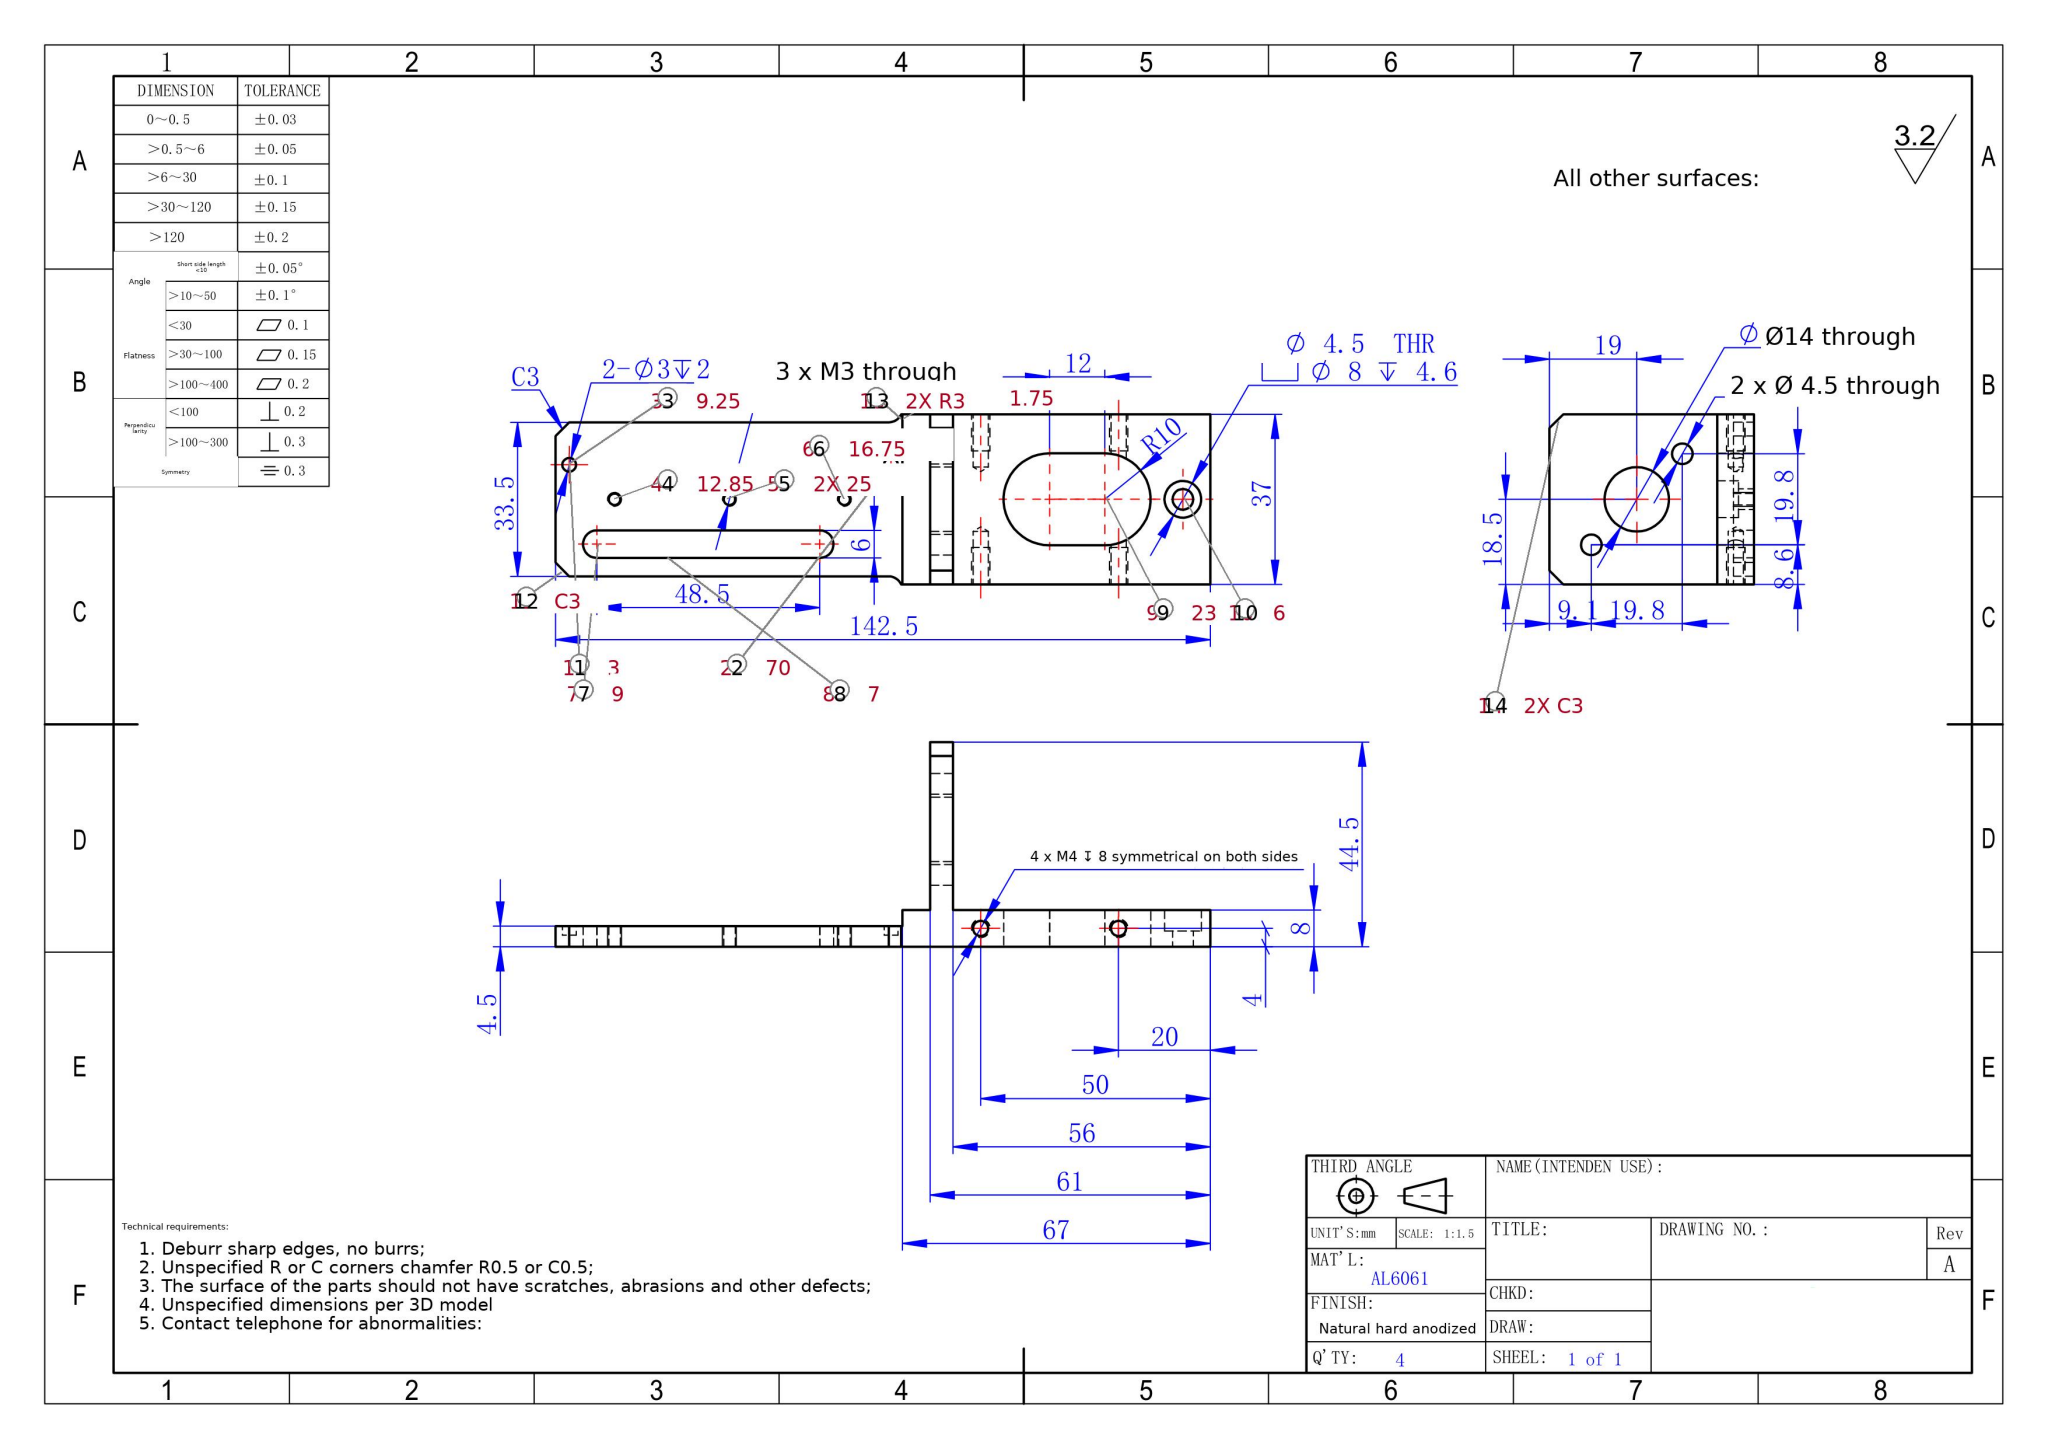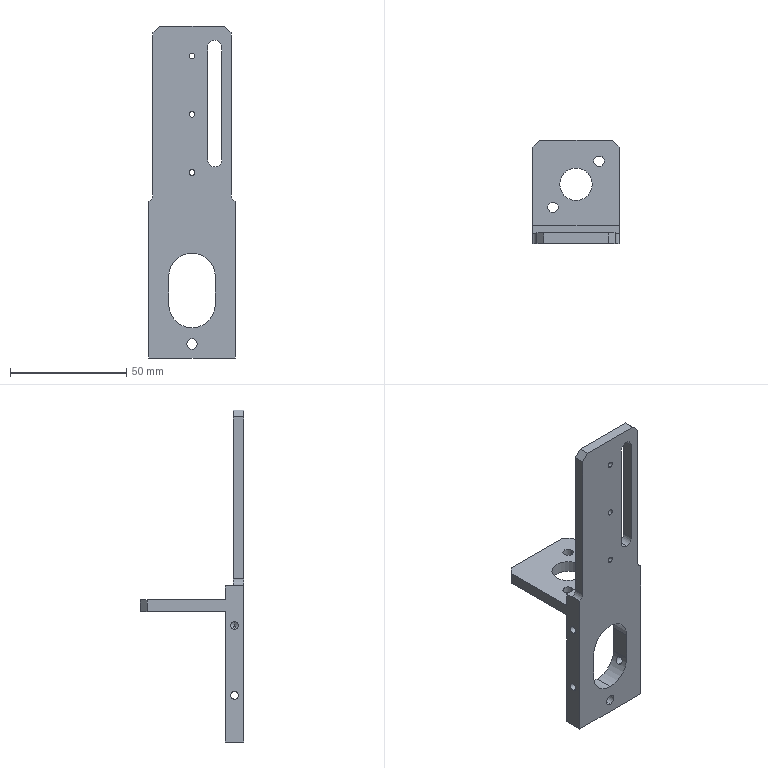Part | SolidWorks | mm | material AL6061 | 1 solid | 65 faces | box 37 x 44.5 x 142.5 mm | volume 30362 mm3 | cylinder 36 | plane 25 | cone 4 | commonest cylinder face diameters 3.3 x8 4.5 x6 2.5 x6 6 x5 3 x4 20 x3 8 x2 14 x2